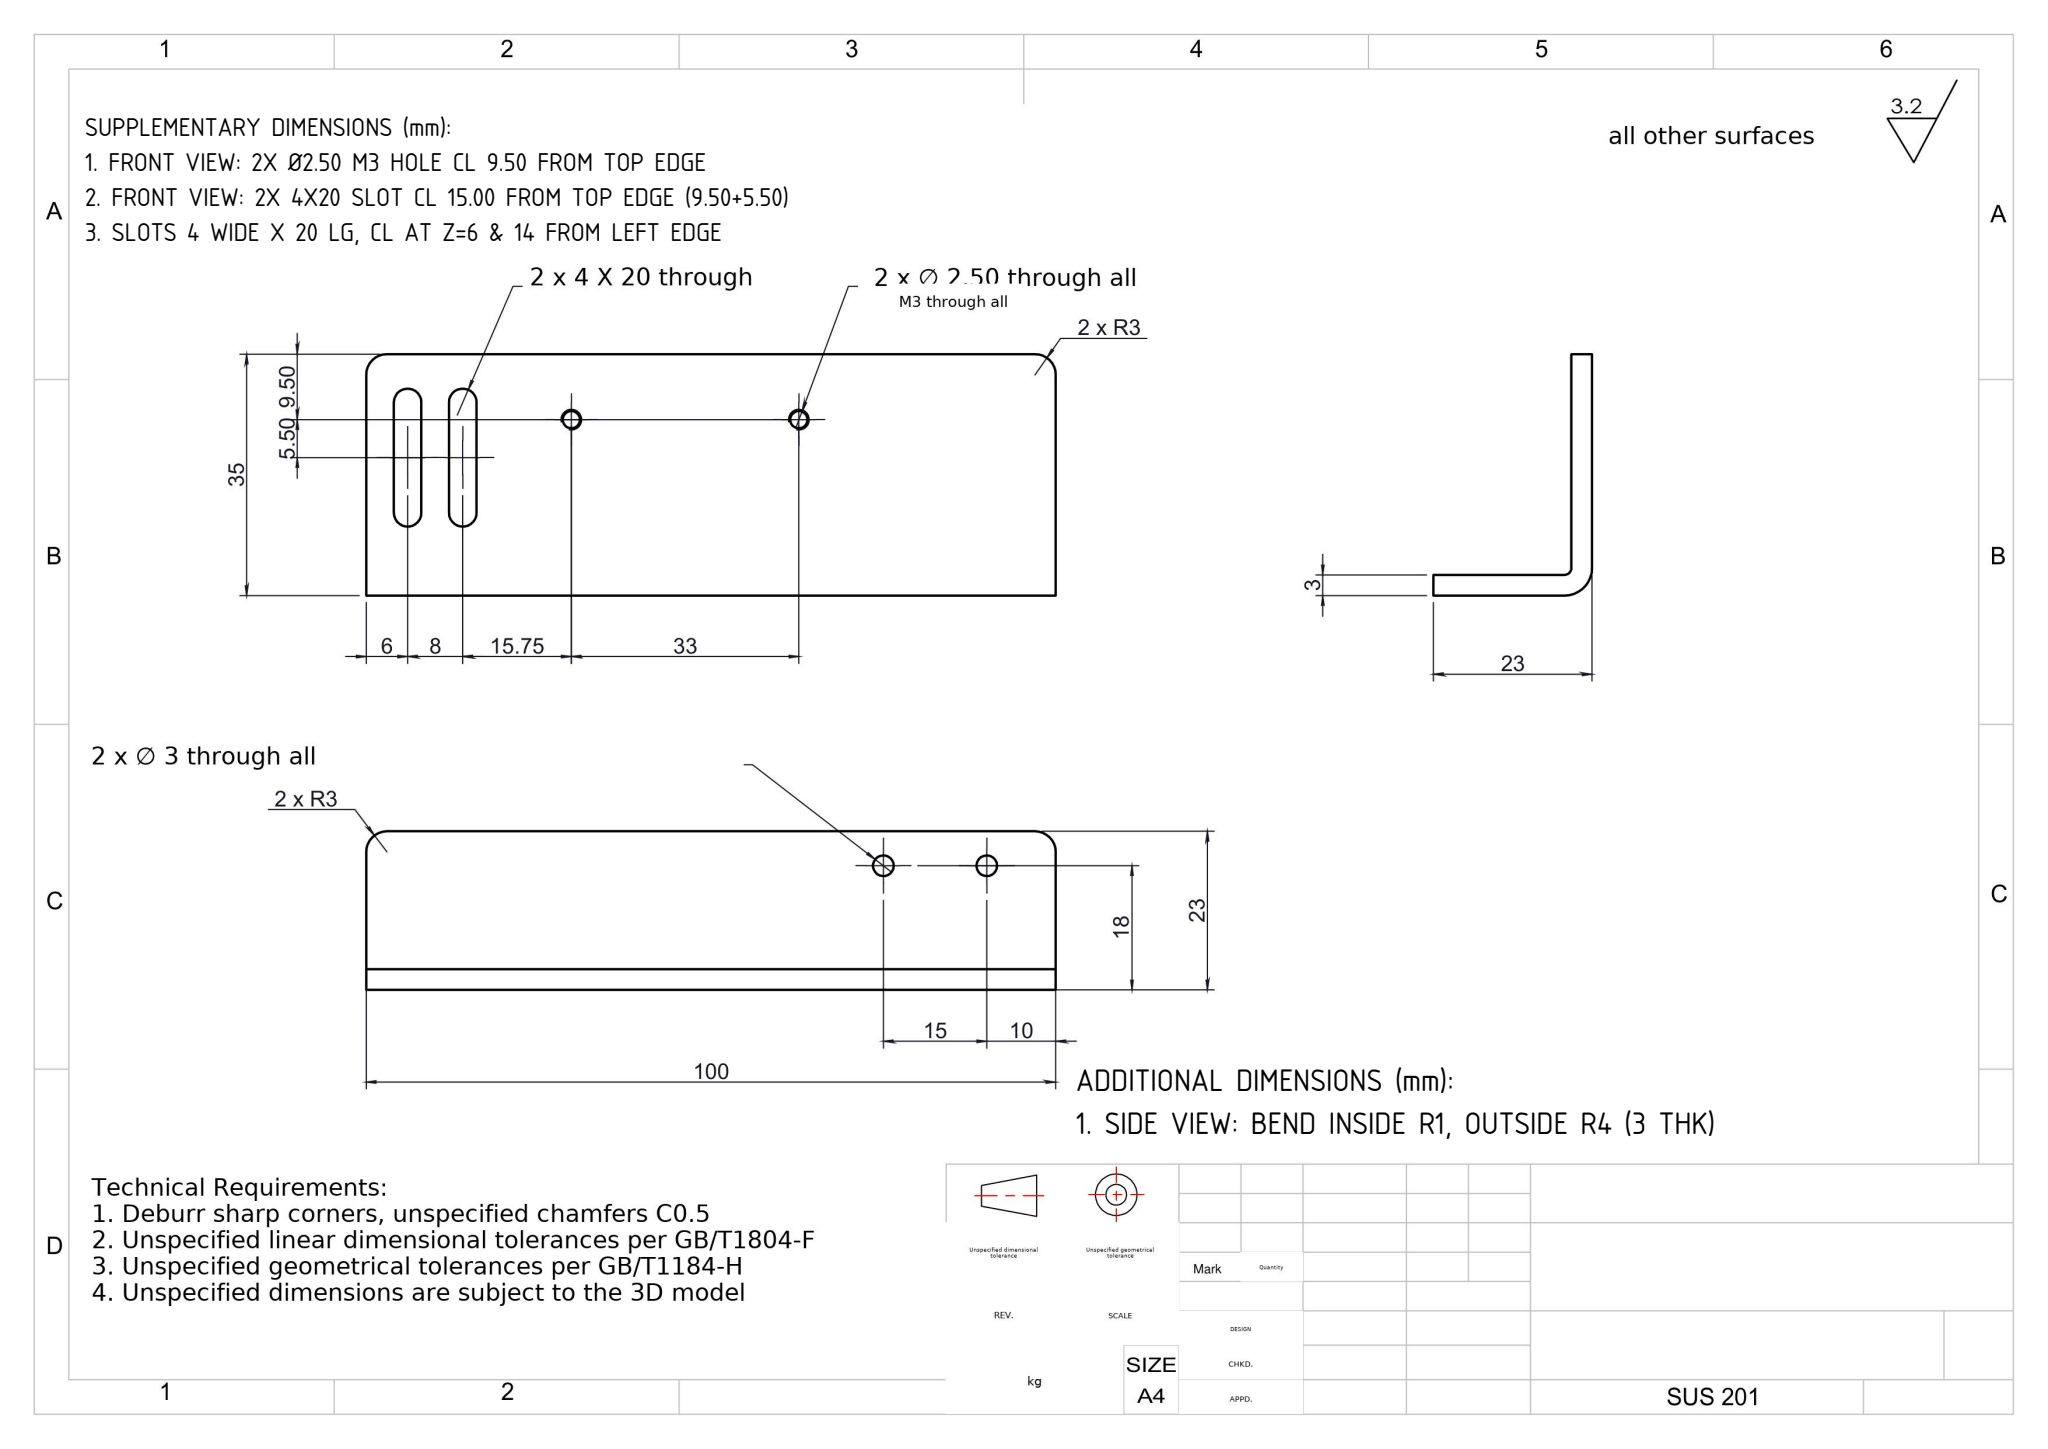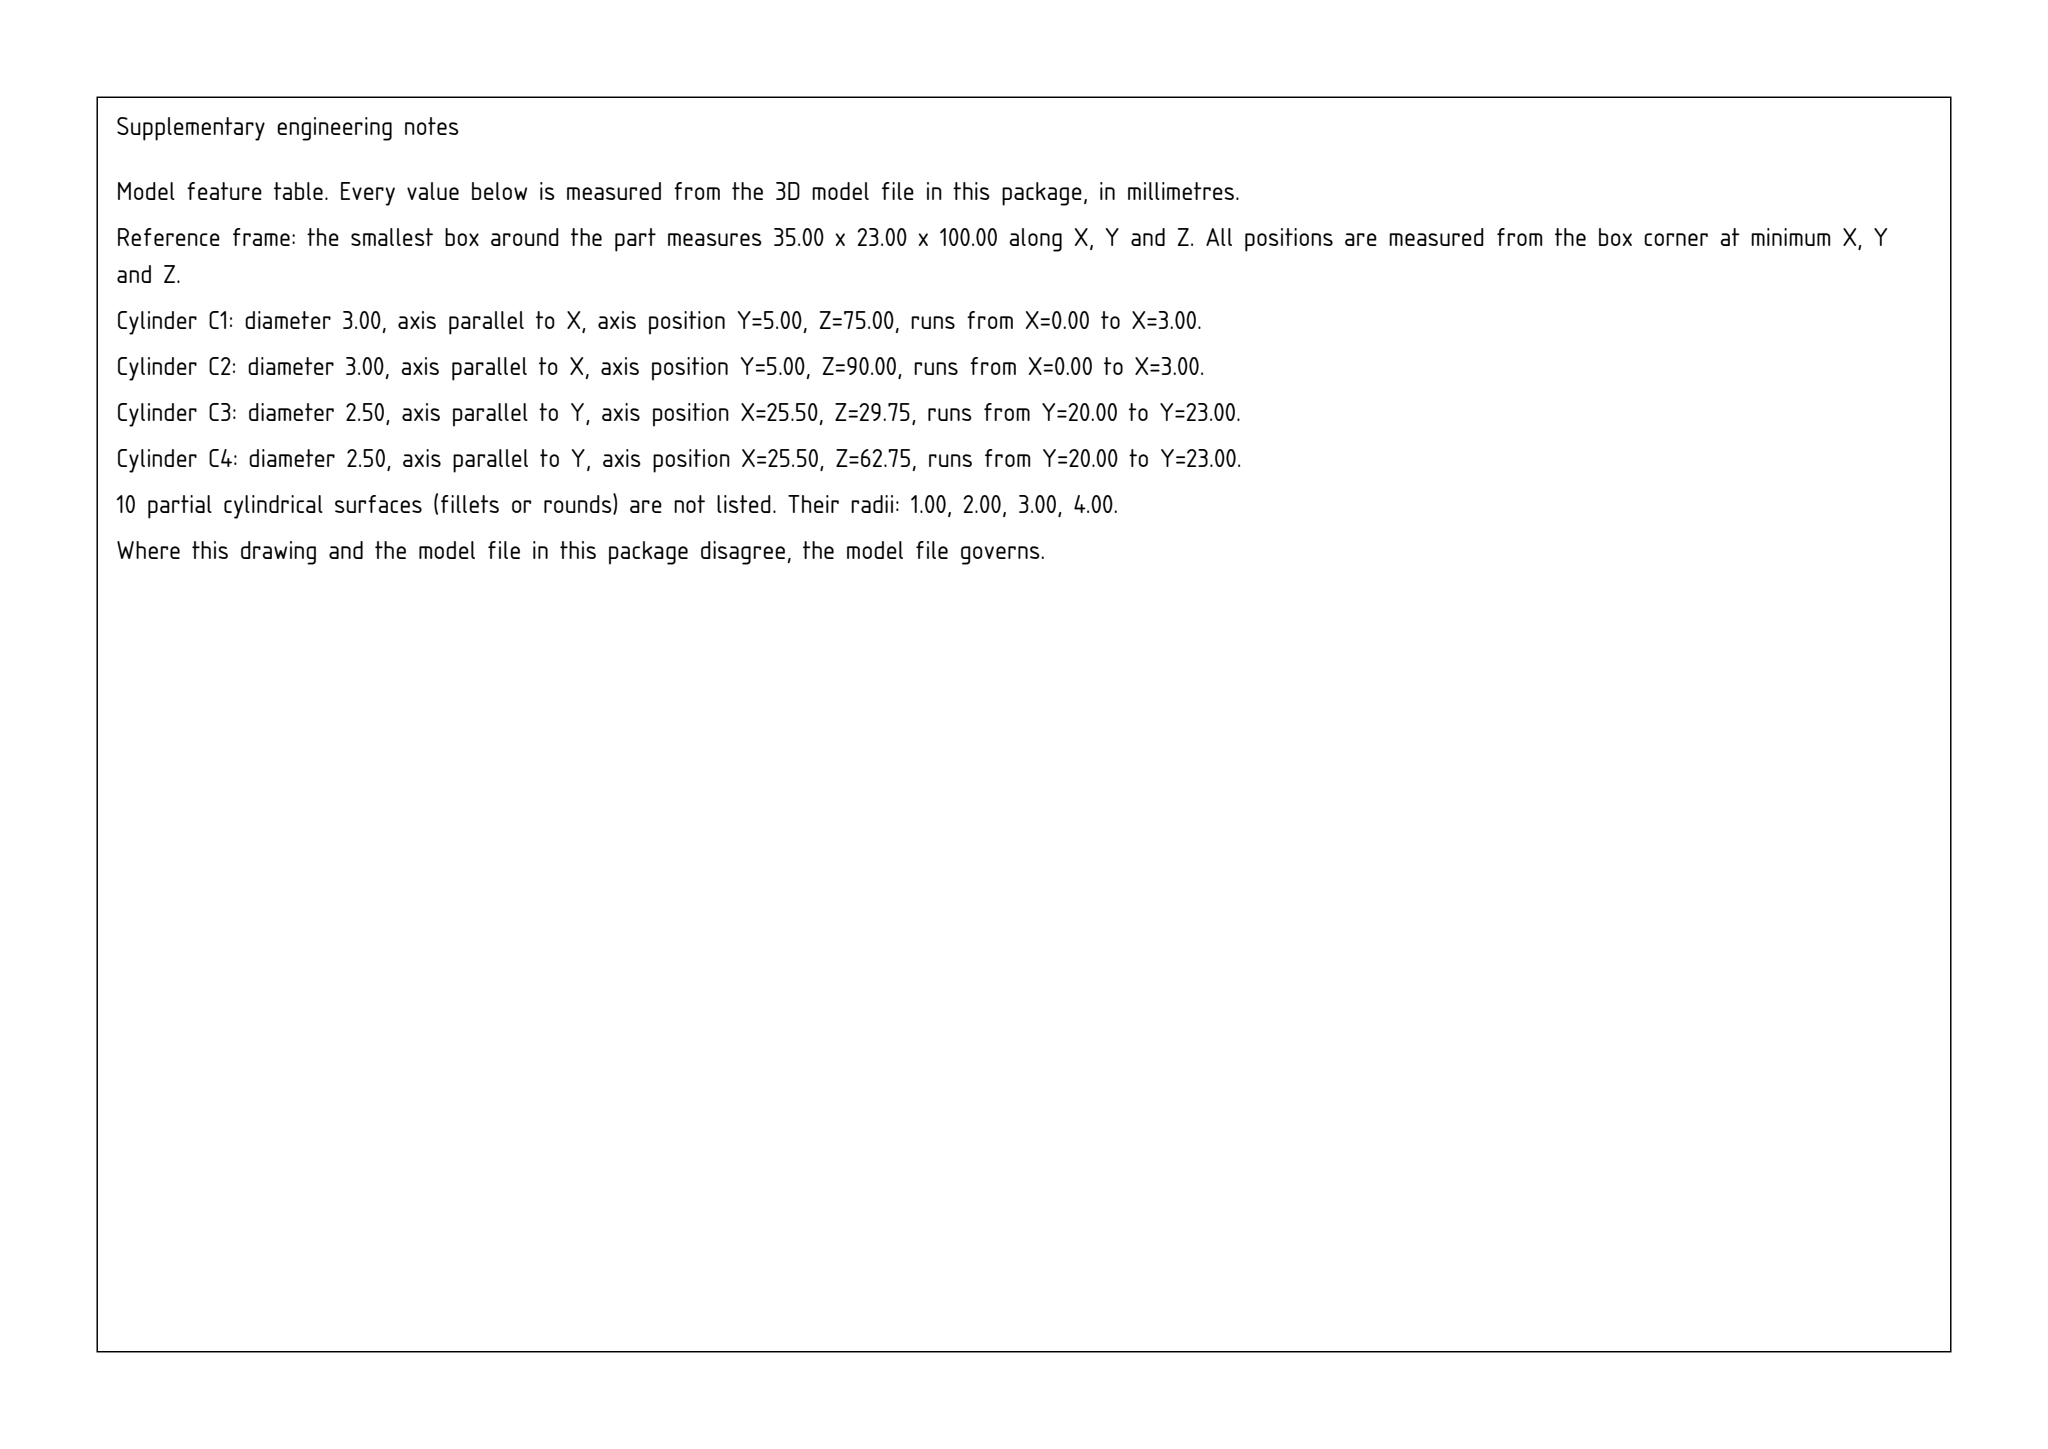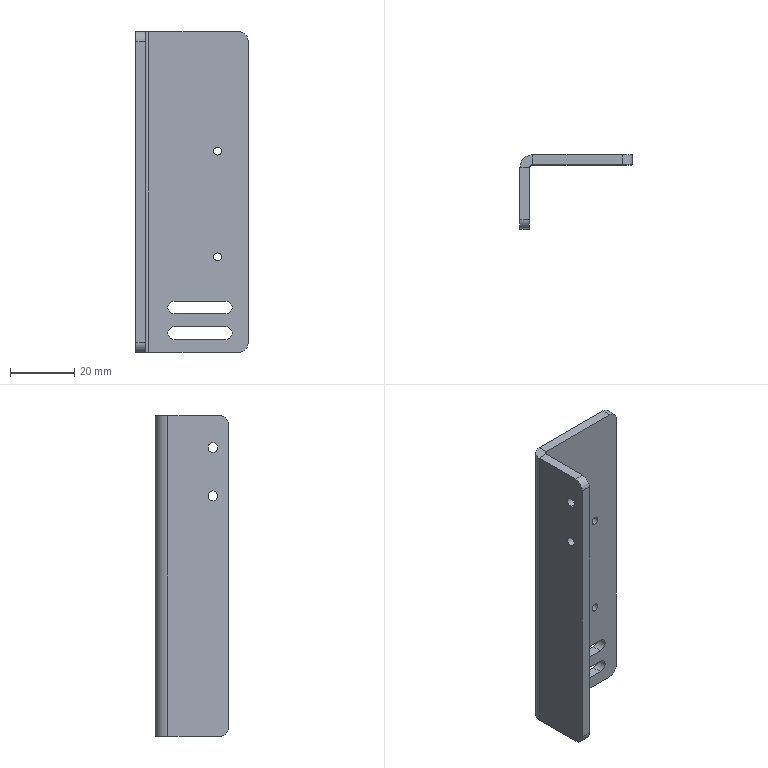Part | SolidWorks | mm | 1 solid | 34 faces | box 35 x 23 x 100 mm | volume 15624 mm3 | cylinder 18 | plane 16 | commonest cylinder face diameters 2.5 x4 3 x4 4 x4 6 x4 8 x1 2 x1